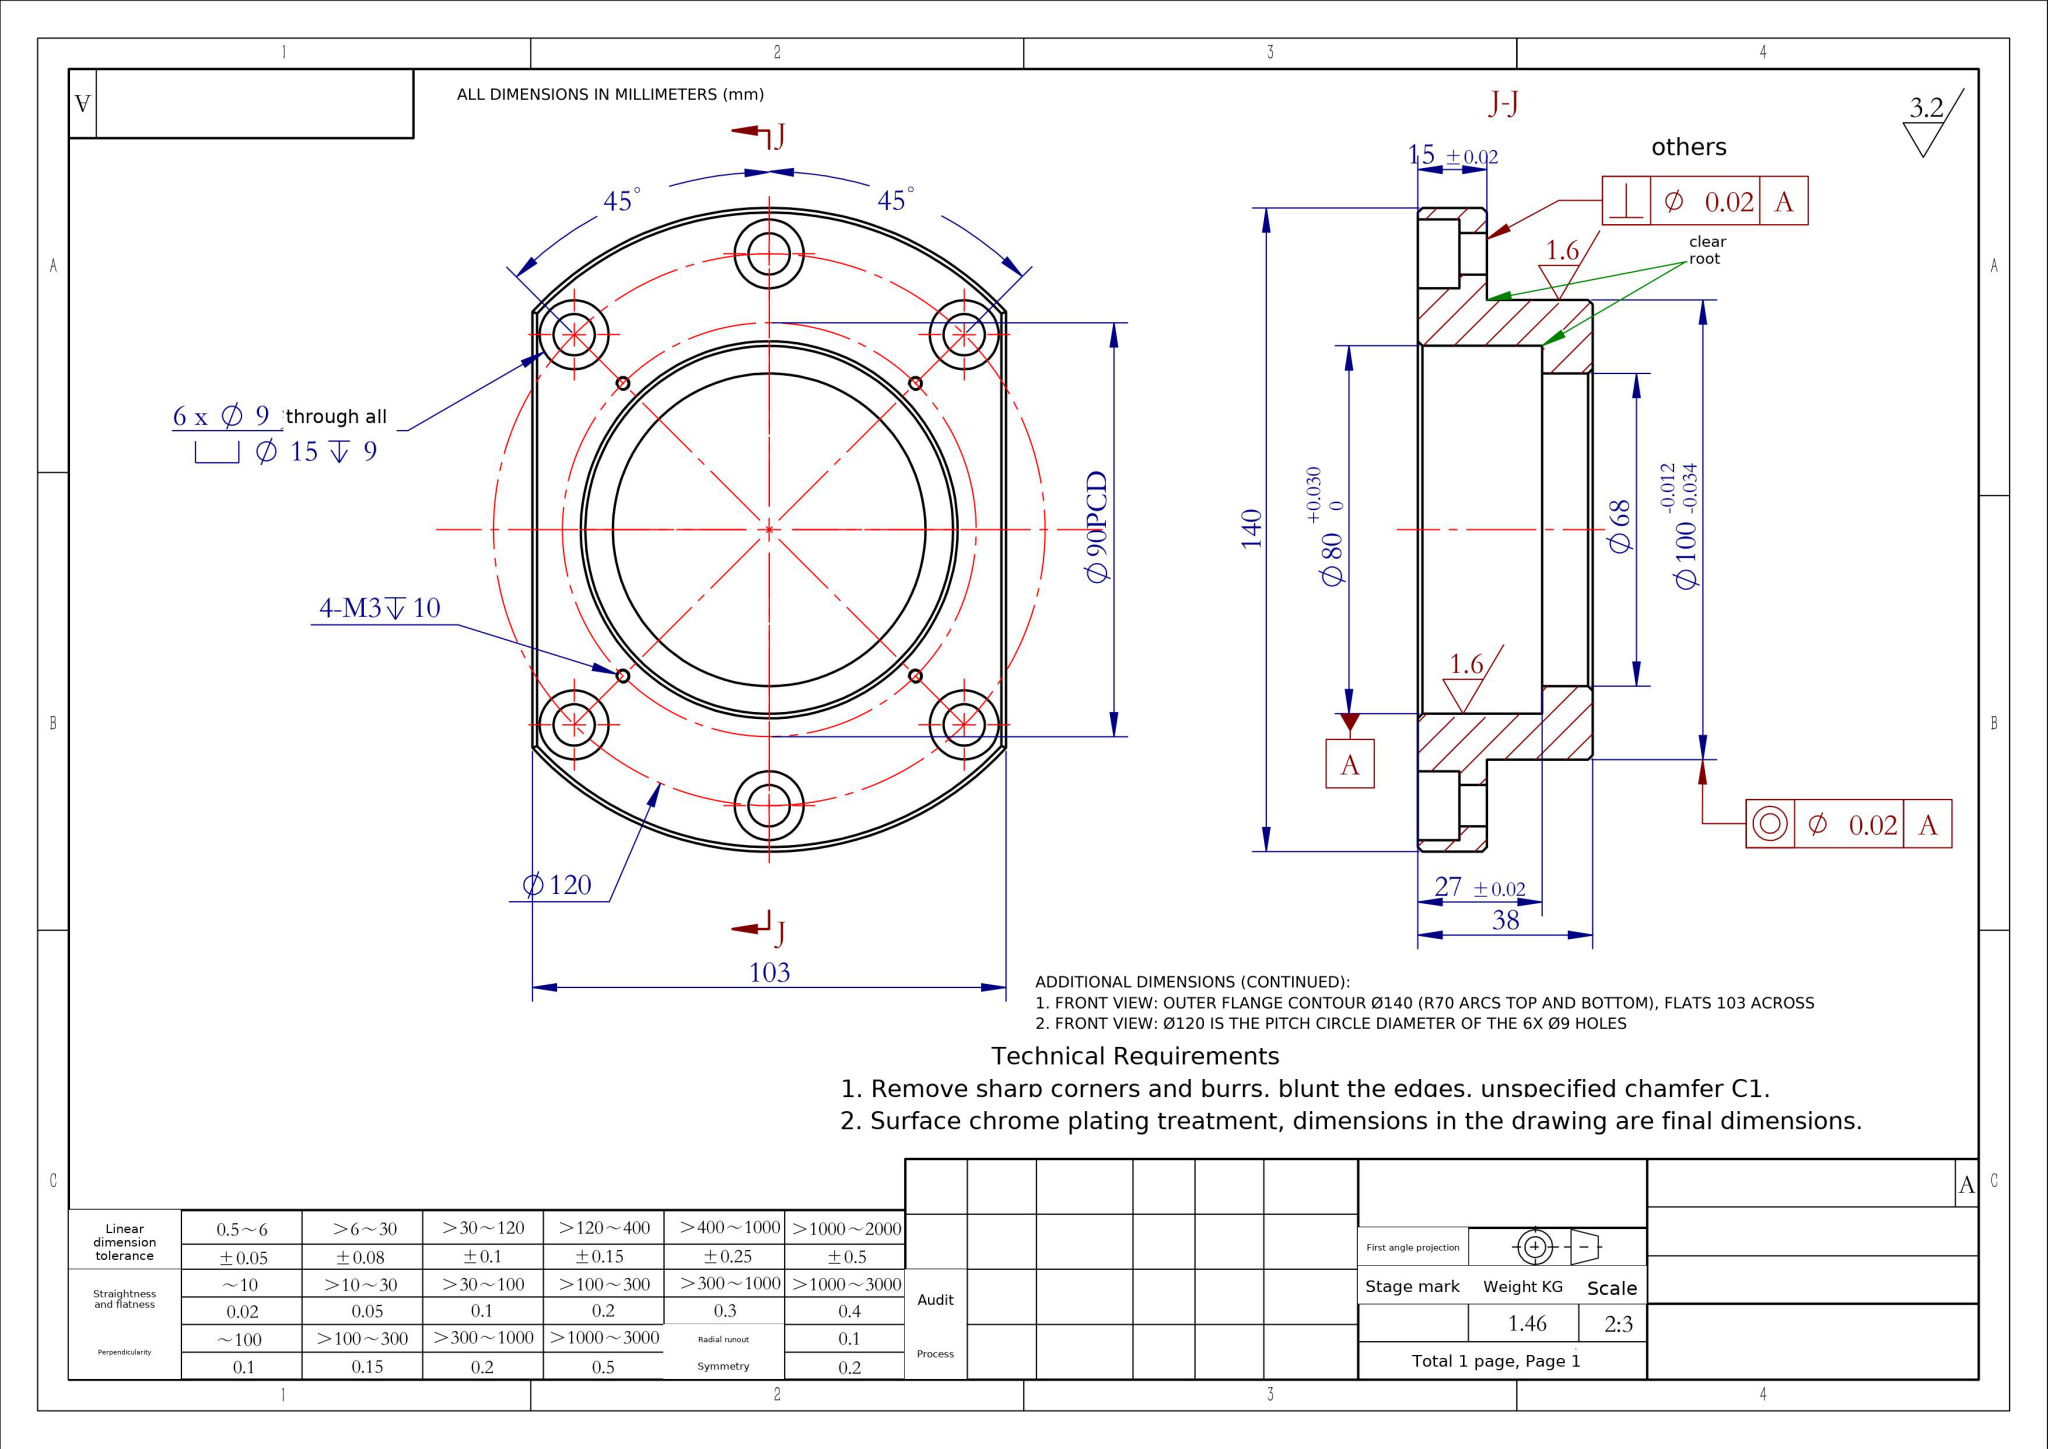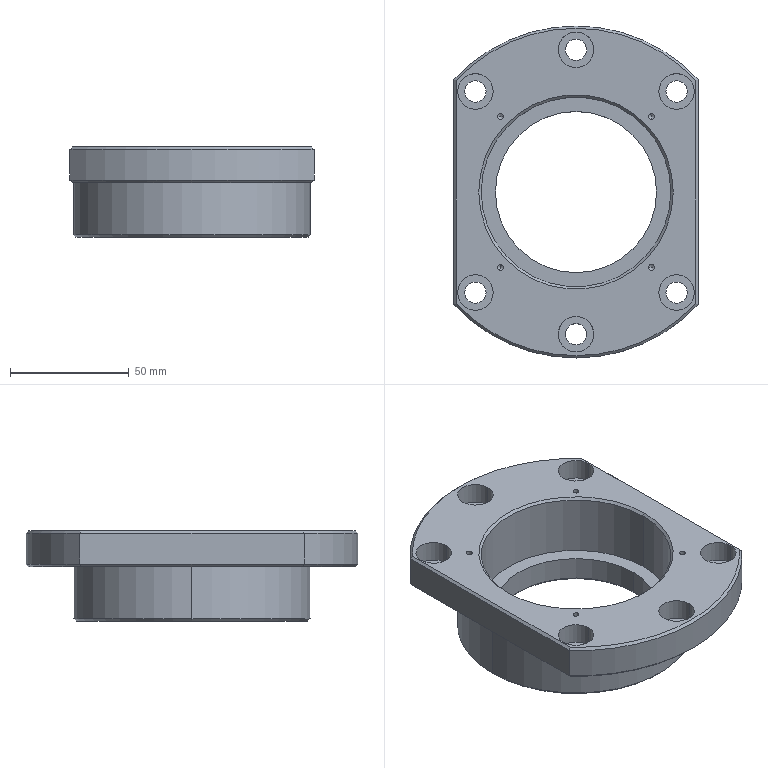Part | NX | mm | 1 solid | 74 faces | box 103 x 140 x 38 mm | volume 186959 mm3 | cylinder 40 | cone 18 | plane 16 | commonest cylinder face diameters 15 x12 9 x12 2.5 x8 68 x2 80 x2 100 x2 140 x2